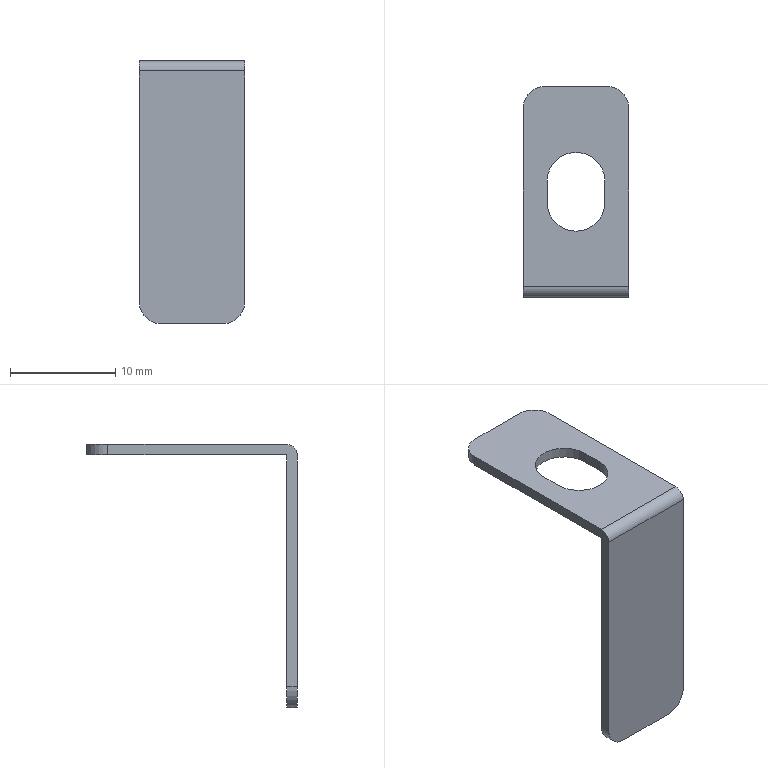Component | SolidWorks | BearingHousingAssembly-1_SensorPlate3-1 | 1 solid | 18 faces | box 10 x 20 x 25 mm | volume 400 mm3 | plane 10 | cylinder 8 | commonest cylinder face diameters 4 x4 5.5 x3 2 x1 | material Plain Carbon Steel
build123d program:
from build123d import *

# Parameters (mm, degrees)
EXTRUDE_THIN1_DEPTH = 5
FILLET1_R           = 1
FILLET2_R           = 2
CUT_EXTRUDE1_DEPTH  = 33.404


with BuildPart() as part:
    # Sketch1 → Extrude-Thin1 (new, symmetric)
    with BuildSketch(Plane.XY):
        Polygon((0, 20), (0, 0), (25, 0), (25, 1), (1, 1), (1, 20), align=None)
    extrude(amount=EXTRUDE_THIN1_DEPTH, both=True)

    # Fillet1
    fillet1_edges = [part.edges().sort_by_distance(p)[0] for p in [
        (0, 0, 0),
    ]]
    fillet(fillet1_edges, radius=FILLET1_R)

    # Fillet2
    fillet2_edges = [part.edges().sort_by_distance(p)[0] for p in [
        (0.5, 20, 5),
        (0.5, 20, -5),
        (25, 0.5, -5),
        (25, 0.5, 5),
    ]]
    fillet(fillet2_edges, radius=FILLET2_R)

    # Sketch2 → Cut-Extrude1 (cut, through all)
    with BuildSketch(Plane.ZY):
        with BuildLine():
            Line((-2.75, 9), (-2.75, 11))
            ThreePointArc((-2.75, 11), (0, 13.75), (2.75, 11))
            Line((2.75, 11), (2.75, 9))
            ThreePointArc((2.75, 9), (0, 6.25), (-2.75, 9))
        make_face()
    extrude(amount=-CUT_EXTRUDE1_DEPTH, mode=Mode.SUBTRACT)


solid = part.part

# Placed as in the assembly
solid = solid.moved(Location((-81.666, 41.264, -46), (0, 90, 0)))
STEP:
#1=COLOUR_RGB('',0.7922,0.8196,0.9333);
#2=FILL_AREA_STYLE_COLOUR('',#1);
#3=FILL_AREA_STYLE('',(#2));
#4=SURFACE_STYLE_FILL_AREA(#3);
#5=SURFACE_SIDE_STYLE('',(#4));
#6=SURFACE_STYLE_USAGE(.BOTH.,#5);
#7=PRESENTATION_STYLE_ASSIGNMENT((#6));
#8=CARTESIAN_POINT('',(-3.107,1.979,-1.85));
#9=VERTEX_POINT('',#8);
#10=CARTESIAN_POINT('',(-3.215,1.871,-1.85));
#11=VERTEX_POINT('',#10);
#12=CARTESIAN_POINT('',(-3.215,1.979,-1.85));
#13=DIRECTION('',(-0.,-0.,-1.));
#14=DIRECTION('',(0.,1.,0.));
#15=AXIS2_PLACEMENT_3D('',#12,#13,#14);
#16=CIRCLE('',#15,0.1083);
#17=EDGE_CURVE('',#9,#11,#16,.T.);
#18=ORIENTED_EDGE('',*,*,#17,.T.);
#19=CARTESIAN_POINT('',(-3.215,1.871,-1.811));
#20=VERTEX_POINT('',#19);
#21=CARTESIAN_POINT('',(-3.215,1.871,-2.795));
#22=DIRECTION('',(0.,0.,1.));
#23=VECTOR('',#22,39.37);
#24=LINE('',#21,#23);
#25=EDGE_CURVE('',#11,#20,#24,.T.);
#26=ORIENTED_EDGE('',*,*,#25,.T.);
#27=CARTESIAN_POINT('',(-3.107,1.979,-1.811));
#28=VERTEX_POINT('',#27);
#29=CARTESIAN_POINT('',(-3.215,1.979,-1.811));
#30=DIRECTION('',(0.,0.,1.));
#31=DIRECTION('',(0.,-1.,0.));
#32=AXIS2_PLACEMENT_3D('',#29,#30,#31);
#33=CIRCLE('',#32,0.1083);
#34=EDGE_CURVE('',#20,#28,#33,.T.);
#35=ORIENTED_EDGE('',*,*,#34,.T.);
#36=CARTESIAN_POINT('',(-3.107,1.979,-2.795));
#37=DIRECTION('',(0.,0.,1.));
#38=VECTOR('',#37,39.37);
#39=LINE('',#36,#38);
#40=EDGE_CURVE('',#9,#28,#39,.T.);
#41=ORIENTED_EDGE('',*,*,#40,.F.);
#42=EDGE_LOOP('',(#18,#26,#35,#41));
#43=FACE_OUTER_BOUND('',#42,.T.);
#44=CARTESIAN_POINT('',(-3.215,1.979,-2.795));
#45=DIRECTION('',(0.,0.,1.));
#46=DIRECTION('',(0.,-1.,0.));
#47=AXIS2_PLACEMENT_3D('',#44,#45,#46);
#48=CYLINDRICAL_SURFACE('',#47,0.1083);
#49=ADVANCED_FACE('',(#43),#48,.F.);
#50=CARTESIAN_POINT('',(-3.412,1.625,-1.85));
#51=VERTEX_POINT('',#50);
#52=CARTESIAN_POINT('',(-3.412,1.625,-2.717));
#53=VERTEX_POINT('',#52);
#54=CARTESIAN_POINT('',(-3.412,1.625,-1.811));
#55=DIRECTION('',(-0.,0.,-1.));
#56=VECTOR('',#55,39.37);
#57=LINE('',#54,#56);
#58=EDGE_CURVE('',#51,#53,#57,.T.);
#59=ORIENTED_EDGE('',*,*,#58,.T.);
#60=CARTESIAN_POINT('',(-3.333,1.625,-2.795));
#61=VERTEX_POINT('',#60);
#62=CARTESIAN_POINT('',(-3.333,1.625,-2.717));
#63=DIRECTION('',(-0.,-1.,-0.));
#64=DIRECTION('',(1.,0.,-0.));
#65=AXIS2_PLACEMENT_3D('',#62,#63,#64);
#66=CIRCLE('',#65,0.07874);
#67=EDGE_CURVE('',#53,#61,#66,.T.);
#68=ORIENTED_EDGE('',*,*,#67,.T.);
#69=CARTESIAN_POINT('',(-3.097,1.625,-2.795));
#70=VERTEX_POINT('',#69);
#71=CARTESIAN_POINT('',(-3.018,1.625,-2.795));
#72=DIRECTION('',(-1.,0.,0.));
#73=VECTOR('',#72,39.37);
#74=LINE('',#71,#73);
#75=EDGE_CURVE('',#70,#61,#74,.T.);
#76=ORIENTED_EDGE('',*,*,#75,.F.);
#77=CARTESIAN_POINT('',(-3.018,1.625,-2.717));
#78=VERTEX_POINT('',#77);
#79=CARTESIAN_POINT('',(-3.097,1.625,-2.717));
#80=DIRECTION('',(-0.,-1.,-0.));
#81=DIRECTION('',(1.,0.,-0.));
#82=AXIS2_PLACEMENT_3D('',#79,#80,#81);
#83=CIRCLE('',#82,0.07874);
#84=EDGE_CURVE('',#70,#78,#83,.T.);
#85=ORIENTED_EDGE('',*,*,#84,.T.);
#86=CARTESIAN_POINT('',(-3.018,1.625,-1.85));
#87=VERTEX_POINT('',#86);
#88=CARTESIAN_POINT('',(-3.018,1.625,-1.811));
#89=DIRECTION('',(-0.,0.,-1.));
#90=VECTOR('',#89,39.37);
#91=LINE('',#88,#90);
#92=EDGE_CURVE('',#87,#78,#91,.T.);
#93=ORIENTED_EDGE('',*,*,#92,.F.);
#94=CARTESIAN_POINT('',(-3.018,1.625,-1.85));
#95=DIRECTION('',(-1.,0.,0.));
#96=VECTOR('',#95,39.37);
#97=LINE('',#94,#96);
#98=EDGE_CURVE('',#87,#51,#97,.T.);
#99=ORIENTED_EDGE('',*,*,#98,.T.);
#100=EDGE_LOOP('',(#59,#68,#76,#85,#93,#99));
#101=FACE_OUTER_BOUND('',#100,.T.);
#102=CARTESIAN_POINT('',(-3.018,1.625,-1.811));
#103=DIRECTION('',(0.,1.,0.));
#104=DIRECTION('',(1.,-0.,-0.));
#105=AXIS2_PLACEMENT_3D('',#102,#103,#104);
#106=PLANE('',#105);
#107=ADVANCED_FACE('',(#101),#106,.F.);
#108=ORIENTED_EDGE('',*,*,#75,.T.);
#109=CARTESIAN_POINT('',(-3.333,1.664,-2.795));
#110=VERTEX_POINT('',#109);
#111=CARTESIAN_POINT('',(-3.333,1.664,-2.795));
#112=DIRECTION('',(0.,1.,0.));
#113=VECTOR('',#112,39.37);
#114=LINE('',#111,#113);
#115=EDGE_CURVE('',#61,#110,#114,.T.);
#116=ORIENTED_EDGE('',*,*,#115,.T.);
#117=CARTESIAN_POINT('',(-3.097,1.664,-2.795));
#118=VERTEX_POINT('',#117);
#119=CARTESIAN_POINT('',(-3.018,1.664,-2.795));
#120=DIRECTION('',(-1.,0.,0.));
#121=VECTOR('',#120,39.37);
#122=LINE('',#119,#121);
#123=EDGE_CURVE('',#118,#110,#122,.T.);
#124=ORIENTED_EDGE('',*,*,#123,.F.);
#125=CARTESIAN_POINT('',(-3.097,1.625,-2.795));
#126=DIRECTION('',(-0.,-1.,-0.));
#127=VECTOR('',#126,39.37);
#128=LINE('',#125,#127);
#129=EDGE_CURVE('',#118,#70,#128,.T.);
#130=ORIENTED_EDGE('',*,*,#129,.T.);
#131=EDGE_LOOP('',(#108,#116,#124,#130));
#132=FACE_OUTER_BOUND('',#131,.T.);
#133=CARTESIAN_POINT('',(-3.018,1.664,-2.795));
#134=DIRECTION('',(-0.,0.,-1.));
#135=DIRECTION('',(-1.,0.,0.));
#136=AXIS2_PLACEMENT_3D('',#133,#134,#135);
#137=PLANE('',#136);
#138=ADVANCED_FACE('',(#132),#137,.T.);
#139=ORIENTED_EDGE('',*,*,#123,.T.);
#140=CARTESIAN_POINT('',(-3.412,1.664,-2.717));
#141=VERTEX_POINT('',#140);
#142=CARTESIAN_POINT('',(-3.333,1.664,-2.717));
#143=DIRECTION('',(0.,1.,0.));
#144=DIRECTION('',(1.,0.,-0.));
#145=AXIS2_PLACEMENT_3D('',#142,#143,#144);
#146=CIRCLE('',#145,0.07874);
#147=EDGE_CURVE('',#110,#141,#146,.T.);
#148=ORIENTED_EDGE('',*,*,#147,.T.);
#149=CARTESIAN_POINT('',(-3.412,1.664,-1.85));
#150=VERTEX_POINT('',#149);
#151=CARTESIAN_POINT('',(-3.412,1.664,-1.811));
#152=DIRECTION('',(-0.,0.,-1.));
#153=VECTOR('',#152,39.37);
#154=LINE('',#151,#153);
#155=EDGE_CURVE('',#150,#141,#154,.T.);
#156=ORIENTED_EDGE('',*,*,#155,.F.);
#157=CARTESIAN_POINT('',(-3.018,1.664,-1.85));
#158=VERTEX_POINT('',#157);
#159=CARTESIAN_POINT('',(-3.018,1.664,-1.85));
#160=DIRECTION('',(-1.,0.,0.));
#161=VECTOR('',#160,39.37);
#162=LINE('',#159,#161);
#163=EDGE_CURVE('',#158,#150,#162,.T.);
#164=ORIENTED_EDGE('',*,*,#163,.F.);
#165=CARTESIAN_POINT('',(-3.018,1.664,-2.717));
#166=VERTEX_POINT('',#165);
#167=CARTESIAN_POINT('',(-3.018,1.664,-1.811));
#168=DIRECTION('',(-0.,0.,-1.));
#169=VECTOR('',#168,39.37);
#170=LINE('',#167,#169);
#171=EDGE_CURVE('',#158,#166,#170,.T.);
#172=ORIENTED_EDGE('',*,*,#171,.T.);
#173=CARTESIAN_POINT('',(-3.097,1.664,-2.717));
#174=DIRECTION('',(0.,1.,0.));
#175=DIRECTION('',(1.,0.,-0.));
#176=AXIS2_PLACEMENT_3D('',#173,#174,#175);
#177=CIRCLE('',#176,0.07874);
#178=EDGE_CURVE('',#166,#118,#177,.T.);
#179=ORIENTED_EDGE('',*,*,#178,.T.);
#180=EDGE_LOOP('',(#139,#148,#156,#164,#172,#179));
#181=FACE_OUTER_BOUND('',#180,.T.);
#182=CARTESIAN_POINT('',(-3.018,1.664,-1.811));
#183=DIRECTION('',(0.,1.,0.));
#184=DIRECTION('',(1.,-0.,-0.));
#185=AXIS2_PLACEMENT_3D('',#182,#183,#184);
#186=PLANE('',#185);
#187=ADVANCED_FACE('',(#181),#186,.T.);
#188=ORIENTED_EDGE('',*,*,#17,.F.);
#189=CARTESIAN_POINT('',(-3.107,2.058,-1.85));
#190=VERTEX_POINT('',#189);
#191=CARTESIAN_POINT('',(-3.107,2.412,-1.85));
#192=DIRECTION('',(0.,-1.,0.));
#193=VECTOR('',#192,39.37);
#194=LINE('',#191,#193);
#195=EDGE_CURVE('',#190,#9,#194,.T.);
#196=ORIENTED_EDGE('',*,*,#195,.F.);
#197=CARTESIAN_POINT('',(-3.323,2.058,-1.85));
#198=VERTEX_POINT('',#197);
#199=CARTESIAN_POINT('',(-3.215,2.058,-1.85));
#200=DIRECTION('',(-0.,-0.,-1.));
#201=DIRECTION('',(0.,1.,0.));
#202=AXIS2_PLACEMENT_3D('',#199,#200,#201);
#203=CIRCLE('',#202,0.1083);
#204=EDGE_CURVE('',#198,#190,#203,.T.);
#205=ORIENTED_EDGE('',*,*,#204,.F.);
#206=CARTESIAN_POINT('',(-3.323,1.979,-1.85));
#207=VERTEX_POINT('',#206);
#208=CARTESIAN_POINT('',(-3.323,2.412,-1.85));
#209=DIRECTION('',(-0.,1.,-0.));
#210=VECTOR('',#209,39.37);
#211=LINE('',#208,#210);
#212=EDGE_CURVE('',#207,#198,#211,.T.);
#213=ORIENTED_EDGE('',*,*,#212,.F.);
#214=CARTESIAN_POINT('',(-3.215,1.979,-1.85));
#215=DIRECTION('',(-0.,-0.,-1.));
#216=DIRECTION('',(0.,1.,0.));
#217=AXIS2_PLACEMENT_3D('',#214,#215,#216);
#218=CIRCLE('',#217,0.1083);
#219=EDGE_CURVE('',#11,#207,#218,.T.);
#220=ORIENTED_EDGE('',*,*,#219,.F.);
#221=EDGE_LOOP('',(#188,#196,#205,#213,#220));
#222=FACE_BOUND('',#221,.T.);
#223=CARTESIAN_POINT('',(-3.412,2.333,-1.85));
#224=VERTEX_POINT('',#223);
#225=CARTESIAN_POINT('',(-3.412,2.412,-1.85));
#226=DIRECTION('',(-0.,-1.,0.));
#227=VECTOR('',#226,39.37);
#228=LINE('',#225,#227);
#229=EDGE_CURVE('',#224,#150,#228,.T.);
#230=ORIENTED_EDGE('',*,*,#229,.F.);
#231=CARTESIAN_POINT('',(-3.333,2.412,-1.85));
#232=VERTEX_POINT('',#231);
#233=CARTESIAN_POINT('',(-3.333,2.333,-1.85));
#234=DIRECTION('',(-0.,-0.,-1.));
#235=DIRECTION('',(0.,1.,0.));
#236=AXIS2_PLACEMENT_3D('',#233,#234,#235);
#237=CIRCLE('',#236,0.07874);
#238=EDGE_CURVE('',#224,#232,#237,.T.);
#239=ORIENTED_EDGE('',*,*,#238,.T.);
#240=CARTESIAN_POINT('',(-3.097,2.412,-1.85));
#241=VERTEX_POINT('',#240);
#242=CARTESIAN_POINT('',(-3.018,2.412,-1.85));
#243=DIRECTION('',(-1.,0.,0.));
#244=VECTOR('',#243,39.37);
#245=LINE('',#242,#244);
#246=EDGE_CURVE('',#241,#232,#245,.T.);
#247=ORIENTED_EDGE('',*,*,#246,.F.);
#248=CARTESIAN_POINT('',(-3.018,2.333,-1.85));
#249=VERTEX_POINT('',#248);
#250=CARTESIAN_POINT('',(-3.097,2.333,-1.85));
#251=DIRECTION('',(-0.,-0.,-1.));
#252=DIRECTION('',(0.,1.,0.));
#253=AXIS2_PLACEMENT_3D('',#250,#251,#252);
#254=CIRCLE('',#253,0.07874);
#255=EDGE_CURVE('',#241,#249,#254,.T.);
#256=ORIENTED_EDGE('',*,*,#255,.T.);
#257=CARTESIAN_POINT('',(-3.018,2.412,-1.85));
#258=DIRECTION('',(-0.,-1.,0.));
#259=VECTOR('',#258,39.37);
#260=LINE('',#257,#259);
#261=EDGE_CURVE('',#249,#158,#260,.T.);
#262=ORIENTED_EDGE('',*,*,#261,.T.);
#263=ORIENTED_EDGE('',*,*,#163,.T.);
#264=EDGE_LOOP('',(#230,#239,#247,#256,#262,#263));
#265=FACE_OUTER_BOUND('',#264,.T.);
#266=CARTESIAN_POINT('',(-3.018,2.412,-1.85));
#267=DIRECTION('',(-0.,-0.,-1.));
#268=DIRECTION('',(0.,1.,-0.));
#269=AXIS2_PLACEMENT_3D('',#266,#267,#268);
#270=PLANE('',#269);
#271=ADVANCED_FACE('',(#222,#265),#270,.T.);
#272=ORIENTED_EDGE('',*,*,#246,.T.);
#273=CARTESIAN_POINT('',(-3.333,2.412,-1.811));
#274=VERTEX_POINT('',#273);
#275=CARTESIAN_POINT('',(-3.333,2.412,-1.811));
#276=DIRECTION('',(0.,-0.,1.));
#277=VECTOR('',#276,39.37);
#278=LINE('',#275,#277);
#279=EDGE_CURVE('',#232,#274,#278,.T.);
#280=ORIENTED_EDGE('',*,*,#279,.T.);
#281=CARTESIAN_POINT('',(-3.097,2.412,-1.811));
#282=VERTEX_POINT('',#281);
#283=CARTESIAN_POINT('',(-3.018,2.412,-1.811));
#284=DIRECTION('',(-1.,0.,0.));
#285=VECTOR('',#284,39.37);
#286=LINE('',#283,#285);
#287=EDGE_CURVE('',#282,#274,#286,.T.);
#288=ORIENTED_EDGE('',*,*,#287,.F.);
#289=CARTESIAN_POINT('',(-3.097,2.412,-1.85));
#290=DIRECTION('',(-0.,0.,-1.));
#291=VECTOR('',#290,39.37);
#292=LINE('',#289,#291);
#293=EDGE_CURVE('',#282,#241,#292,.T.);
#294=ORIENTED_EDGE('',*,*,#293,.T.);
#295=EDGE_LOOP('',(#272,#280,#288,#294));
#296=FACE_OUTER_BOUND('',#295,.T.);
#297=CARTESIAN_POINT('',(-3.018,2.412,-1.811));
#298=DIRECTION('',(0.,1.,0.));
#299=DIRECTION('',(1.,-0.,-0.));
#300=AXIS2_PLACEMENT_3D('',#297,#298,#299);
#301=PLANE('',#300);
#302=ADVANCED_FACE('',(#296),#301,.T.);
#303=CARTESIAN_POINT('',(-3.107,2.058,-1.811));
#304=VERTEX_POINT('',#303);
#305=CARTESIAN_POINT('',(-3.107,1.979,-1.811));
#306=DIRECTION('',(-0.,1.,-0.));
#307=VECTOR('',#306,39.37);
#308=LINE('',#305,#307);
#309=EDGE_CURVE('',#28,#304,#308,.T.);
#310=ORIENTED_EDGE('',*,*,#309,.F.);
#311=ORIENTED_EDGE('',*,*,#34,.F.);
#312=CARTESIAN_POINT('',(-3.323,1.979,-1.811));
#313=VERTEX_POINT('',#312);
#314=CARTESIAN_POINT('',(-3.215,1.979,-1.811));
#315=DIRECTION('',(0.,0.,1.));
#316=DIRECTION('',(0.,-1.,0.));
#317=AXIS2_PLACEMENT_3D('',#314,#315,#316);
#318=CIRCLE('',#317,0.1083);
#319=EDGE_CURVE('',#313,#20,#318,.T.);
#320=ORIENTED_EDGE('',*,*,#319,.F.);
#321=CARTESIAN_POINT('',(-3.323,2.058,-1.811));
#322=VERTEX_POINT('',#321);
#323=CARTESIAN_POINT('',(-3.323,1.979,-1.811));
#324=DIRECTION('',(0.,-1.,0.));
#325=VECTOR('',#324,39.37);
#326=LINE('',#323,#325);
#327=EDGE_CURVE('',#322,#313,#326,.T.);
#328=ORIENTED_EDGE('',*,*,#327,.F.);
#329=CARTESIAN_POINT('',(-3.215,2.058,-1.811));
#330=DIRECTION('',(0.,0.,1.));
#331=DIRECTION('',(0.,-1.,0.));
#332=AXIS2_PLACEMENT_3D('',#329,#330,#331);
#333=CIRCLE('',#332,0.1083);
#334=EDGE_CURVE('',#304,#322,#333,.T.);
#335=ORIENTED_EDGE('',*,*,#334,.F.);
#336=EDGE_LOOP('',(#310,#311,#320,#328,#335));
#337=FACE_BOUND('',#336,.T.);
#338=ORIENTED_EDGE('',*,*,#287,.T.);
#339=CARTESIAN_POINT('',(-3.412,2.333,-1.811));
#340=VERTEX_POINT('',#339);
#341=CARTESIAN_POINT('',(-3.333,2.333,-1.811));
#342=DIRECTION('',(0.,0.,1.));
#343=DIRECTION('',(0.,1.,0.));
#344=AXIS2_PLACEMENT_3D('',#341,#342,#343);
#345=CIRCLE('',#344,0.07874);
#346=EDGE_CURVE('',#274,#340,#345,.T.);
#347=ORIENTED_EDGE('',*,*,#346,.T.);
#348=CARTESIAN_POINT('',(-3.412,1.664,-1.811));
#349=VERTEX_POINT('',#348);
#350=CARTESIAN_POINT('',(-3.412,2.412,-1.811));
#351=DIRECTION('',(-0.,-1.,0.));
#352=VECTOR('',#351,39.37);
#353=LINE('',#350,#352);
#354=EDGE_CURVE('',#340,#349,#353,.T.);
#355=ORIENTED_EDGE('',*,*,#354,.T.);
#356=CARTESIAN_POINT('',(-3.018,1.664,-1.811));
#357=VERTEX_POINT('',#356);
#358=CARTESIAN_POINT('',(-3.018,1.664,-1.811));
#359=DIRECTION('',(1.,-0.,-0.));
#360=VECTOR('',#359,39.37);
#361=LINE('',#358,#360);
#362=EDGE_CURVE('',#349,#357,#361,.T.);
#363=ORIENTED_EDGE('',*,*,#362,.T.);
#364=CARTESIAN_POINT('',(-3.018,2.333,-1.811));
#365=VERTEX_POINT('',#364);
#366=CARTESIAN_POINT('',(-3.018,2.412,-1.811));
#367=DIRECTION('',(-0.,-1.,0.));
#368=VECTOR('',#367,39.37);
#369=LINE('',#366,#368);
#370=EDGE_CURVE('',#365,#357,#369,.T.);
#371=ORIENTED_EDGE('',*,*,#370,.F.);
#372=CARTESIAN_POINT('',(-3.097,2.333,-1.811));
#373=DIRECTION('',(0.,0.,1.));
#374=DIRECTION('',(0.,1.,0.));
#375=AXIS2_PLACEMENT_3D('',#372,#373,#374);
#376=CIRCLE('',#375,0.07874);
#377=EDGE_CURVE('',#365,#282,#376,.T.);
#378=ORIENTED_EDGE('',*,*,#377,.T.);
#379=EDGE_LOOP('',(#338,#347,#355,#363,#371,#378));
#380=FACE_OUTER_BOUND('',#379,.T.);
#381=CARTESIAN_POINT('',(-3.018,2.412,-1.811));
#382=DIRECTION('',(-0.,-0.,-1.));
#383=DIRECTION('',(0.,1.,-0.));
#384=AXIS2_PLACEMENT_3D('',#381,#382,#383);
#385=PLANE('',#384);
#386=ADVANCED_FACE('',(#337,#380),#385,.F.);
#387=ORIENTED_EDGE('',*,*,#261,.F.);
#388=CARTESIAN_POINT('',(-3.018,2.333,-1.811));
#389=DIRECTION('',(0.,-0.,1.));
#390=VECTOR('',#389,39.37);
#391=LINE('',#388,#390);
#392=EDGE_CURVE('',#249,#365,#391,.T.);
#393=ORIENTED_EDGE('',*,*,#392,.T.);
#394=ORIENTED_EDGE('',*,*,#370,.T.);
#395=CARTESIAN_POINT('',(-3.018,1.664,-1.85));
#396=DIRECTION('',(1.,-0.,-0.));
#397=DIRECTION('',(0.,0.,1.));
#398=AXIS2_PLACEMENT_3D('',#395,#396,#397);
#399=CIRCLE('',#398,0.03937);
#400=EDGE_CURVE('',#357,#87,#399,.T.);
#401=ORIENTED_EDGE('',*,*,#400,.T.);
#402=ORIENTED_EDGE('',*,*,#92,.T.);
#403=CARTESIAN_POINT('',(-3.018,1.664,-2.717));
#404=DIRECTION('',(0.,1.,0.));
#405=VECTOR('',#404,39.37);
#406=LINE('',#403,#405);
#407=EDGE_CURVE('',#78,#166,#406,.T.);
#408=ORIENTED_EDGE('',*,*,#407,.T.);
#409=ORIENTED_EDGE('',*,*,#171,.F.);
#410=EDGE_LOOP('',(#387,#393,#394,#401,#402,#408,#409));
#411=FACE_OUTER_BOUND('',#410,.T.);
#412=CARTESIAN_POINT('',(-3.018,1.625,-1.811));
#413=DIRECTION('',(-1.,0.,0.));
#414=DIRECTION('',(0.,-0.,1.));
#415=AXIS2_PLACEMENT_3D('',#412,#413,#414);
#416=PLANE('',#415);
#417=ADVANCED_FACE('',(#411),#416,.F.);
#418=ORIENTED_EDGE('',*,*,#354,.F.);
#419=CARTESIAN_POINT('',(-3.412,2.333,-1.811));
#420=DIRECTION('',(-0.,0.,-1.));
#421=VECTOR('',#420,39.37);
#422=LINE('',#419,#421);
#423=EDGE_CURVE('',#340,#224,#422,.T.);
#424=ORIENTED_EDGE('',*,*,#423,.T.);
#425=ORIENTED_EDGE('',*,*,#229,.T.);
#426=ORIENTED_EDGE('',*,*,#155,.T.);
#427=CARTESIAN_POINT('',(-3.412,1.625,-2.717));
#428=DIRECTION('',(-0.,-1.,-0.));
#429=VECTOR('',#428,39.37);
#430=LINE('',#427,#429);
#431=EDGE_CURVE('',#141,#53,#430,.T.);
#432=ORIENTED_EDGE('',*,*,#431,.T.);
#433=ORIENTED_EDGE('',*,*,#58,.F.);
#434=CARTESIAN_POINT('',(-3.412,1.664,-1.85));
#435=DIRECTION('',(-1.,0.,0.));
#436=DIRECTION('',(0.,0.,1.));
#437=AXIS2_PLACEMENT_3D('',#434,#435,#436);
#438=CIRCLE('',#437,0.03937);
#439=EDGE_CURVE('',#51,#349,#438,.T.);
#440=ORIENTED_EDGE('',*,*,#439,.T.);
#441=EDGE_LOOP('',(#418,#424,#425,#426,#432,#433,#440));
#442=FACE_OUTER_BOUND('',#441,.T.);
#443=CARTESIAN_POINT('',(-3.412,1.625,-1.811));
#444=DIRECTION('',(-1.,0.,0.));
#445=DIRECTION('',(0.,-0.,1.));
#446=AXIS2_PLACEMENT_3D('',#443,#444,#445);
#447=PLANE('',#446);
#448=ADVANCED_FACE('',(#442),#447,.T.);
#449=ORIENTED_EDGE('',*,*,#400,.F.);
#450=ORIENTED_EDGE('',*,*,#362,.F.);
#451=ORIENTED_EDGE('',*,*,#439,.F.);
#452=ORIENTED_EDGE('',*,*,#98,.F.);
#453=EDGE_LOOP('',(#449,#450,#451,#452));
#454=FACE_OUTER_BOUND('',#453,.T.);
#455=CARTESIAN_POINT('',(-3.018,1.664,-1.85));
#456=DIRECTION('',(-1.,0.,0.));
#457=DIRECTION('',(0.,0.,1.));
#458=AXIS2_PLACEMENT_3D('',#455,#456,#457);
#459=CYLINDRICAL_SURFACE('',#458,0.03937);
#460=ADVANCED_FACE('',(#454),#459,.T.);
#461=ORIENTED_EDGE('',*,*,#346,.F.);
#462=ORIENTED_EDGE('',*,*,#279,.F.);
#463=ORIENTED_EDGE('',*,*,#238,.F.);
#464=ORIENTED_EDGE('',*,*,#423,.F.);
#465=EDGE_LOOP('',(#461,#462,#463,#464));
#466=FACE_OUTER_BOUND('',#465,.T.);
#467=CARTESIAN_POINT('',(-3.333,2.333,-1.811));
#468=DIRECTION('',(-0.,0.,-1.));
#469=DIRECTION('',(-1.,0.,0.));
#470=AXIS2_PLACEMENT_3D('',#467,#468,#469);
#471=CYLINDRICAL_SURFACE('',#470,0.07874);
#472=ADVANCED_FACE('',(#466),#471,.T.);
#473=ORIENTED_EDGE('',*,*,#377,.F.);
#474=ORIENTED_EDGE('',*,*,#392,.F.);
#475=ORIENTED_EDGE('',*,*,#255,.F.);
#476=ORIENTED_EDGE('',*,*,#293,.F.);
#477=EDGE_LOOP('',(#473,#474,#475,#476));
#478=FACE_OUTER_BOUND('',#477,.T.);
#479=CARTESIAN_POINT('',(-3.097,2.333,-1.811));
#480=DIRECTION('',(0.,-0.,1.));
#481=DIRECTION('',(1.,0.,-0.));
#482=AXIS2_PLACEMENT_3D('',#479,#480,#481);
#483=CYLINDRICAL_SURFACE('',#482,0.07874);
#484=ADVANCED_FACE('',(#478),#483,.T.);
#485=ORIENTED_EDGE('',*,*,#147,.F.);
#486=ORIENTED_EDGE('',*,*,#115,.F.);
#487=ORIENTED_EDGE('',*,*,#67,.F.);
#488=ORIENTED_EDGE('',*,*,#431,.F.);
#489=EDGE_LOOP('',(#485,#486,#487,#488));
#490=FACE_OUTER_BOUND('',#489,.T.);
#491=CARTESIAN_POINT('',(-3.333,1.625,-2.717));
#492=DIRECTION('',(-0.,-1.,-0.));
#493=DIRECTION('',(-1.,0.,0.));
#494=AXIS2_PLACEMENT_3D('',#491,#492,#493);
#495=CYLINDRICAL_SURFACE('',#494,0.07874);
#496=ADVANCED_FACE('',(#490),#495,.T.);
#497=ORIENTED_EDGE('',*,*,#178,.F.);
#498=ORIENTED_EDGE('',*,*,#407,.F.);
#499=ORIENTED_EDGE('',*,*,#84,.F.);
#500=ORIENTED_EDGE('',*,*,#129,.F.);
#501=EDGE_LOOP('',(#497,#498,#499,#500));
#502=FACE_OUTER_BOUND('',#501,.T.);
#503=CARTESIAN_POINT('',(-3.097,1.664,-2.717));
#504=DIRECTION('',(0.,1.,0.));
#505=DIRECTION('',(1.,0.,-0.));
#506=AXIS2_PLACEMENT_3D('',#503,#504,#505);
#507=CYLINDRICAL_SURFACE('',#506,0.07874);
#508=ADVANCED_FACE('',(#502),#507,.T.);
#509=ORIENTED_EDGE('',*,*,#25,.F.);
#510=ORIENTED_EDGE('',*,*,#219,.T.);
#511=CARTESIAN_POINT('',(-3.323,1.979,-2.795));
#512=DIRECTION('',(0.,0.,1.));
#513=VECTOR('',#512,39.37);
#514=LINE('',#511,#513);
#515=EDGE_CURVE('',#207,#313,#514,.T.);
#516=ORIENTED_EDGE('',*,*,#515,.T.);
#517=ORIENTED_EDGE('',*,*,#319,.T.);
#518=EDGE_LOOP('',(#509,#510,#516,#517));
#519=FACE_OUTER_BOUND('',#518,.T.);
#520=CARTESIAN_POINT('',(-3.215,1.979,-2.795));
#521=DIRECTION('',(0.,0.,1.));
#522=DIRECTION('',(0.,-1.,0.));
#523=AXIS2_PLACEMENT_3D('',#520,#521,#522);
#524=CYLINDRICAL_SURFACE('',#523,0.1083);
#525=ADVANCED_FACE('',(#519),#524,.F.);
#526=ORIENTED_EDGE('',*,*,#212,.T.);
#527=CARTESIAN_POINT('',(-3.323,2.058,-2.795));
#528=DIRECTION('',(0.,0.,1.));
#529=VECTOR('',#528,39.37);
#530=LINE('',#527,#529);
#531=EDGE_CURVE('',#198,#322,#530,.T.);
#532=ORIENTED_EDGE('',*,*,#531,.T.);
#533=ORIENTED_EDGE('',*,*,#327,.T.);
#534=ORIENTED_EDGE('',*,*,#515,.F.);
#535=EDGE_LOOP('',(#526,#532,#533,#534));
#536=FACE_OUTER_BOUND('',#535,.T.);
#537=CARTESIAN_POINT('',(-3.323,1.979,-2.795));
#538=DIRECTION('',(-1.,-0.,0.));
#539=DIRECTION('',(-0.,1.,0.));
#540=AXIS2_PLACEMENT_3D('',#537,#538,#539);
#541=PLANE('',#540);
#542=ADVANCED_FACE('',(#536),#541,.F.);
#543=ORIENTED_EDGE('',*,*,#204,.T.);
#544=CARTESIAN_POINT('',(-3.107,2.058,-2.795));
#545=DIRECTION('',(0.,0.,1.));
#546=VECTOR('',#545,39.37);
#547=LINE('',#544,#546);
#548=EDGE_CURVE('',#190,#304,#547,.T.);
#549=ORIENTED_EDGE('',*,*,#548,.T.);
#550=ORIENTED_EDGE('',*,*,#334,.T.);
#551=ORIENTED_EDGE('',*,*,#531,.F.);
#552=EDGE_LOOP('',(#543,#549,#550,#551));
#553=FACE_OUTER_BOUND('',#552,.T.);
#554=CARTESIAN_POINT('',(-3.215,2.058,-2.795));
#555=DIRECTION('',(0.,0.,1.));
#556=DIRECTION('',(0.,-1.,0.));
#557=AXIS2_PLACEMENT_3D('',#554,#555,#556);
#558=CYLINDRICAL_SURFACE('',#557,0.1083);
#559=ADVANCED_FACE('',(#553),#558,.F.);
#560=ORIENTED_EDGE('',*,*,#195,.T.);
#561=ORIENTED_EDGE('',*,*,#40,.T.);
#562=ORIENTED_EDGE('',*,*,#309,.T.);
#563=ORIENTED_EDGE('',*,*,#548,.F.);
#564=EDGE_LOOP('',(#560,#561,#562,#563));
#565=FACE_OUTER_BOUND('',#564,.T.);
#566=CARTESIAN_POINT('',(-3.107,1.979,-2.795));
#567=DIRECTION('',(1.,0.,-0.));
#568=DIRECTION('',(0.,-1.,-0.));
#569=AXIS2_PLACEMENT_3D('',#566,#567,#568);
#570=PLANE('',#569);
#571=ADVANCED_FACE('',(#565),#570,.F.);
#572=CLOSED_SHELL('',(#49,#107,#138,#187,#271,#302,#386,#417,#448,#460,#472,#484,#496,#508,#525,#542,#559,#571));
#573=MANIFOLD_SOLID_BREP('',#572);
#574=STYLED_ITEM('',(#7),#573);
#575=(LENGTH_UNIT()NAMED_UNIT(*)SI_UNIT($,.METRE.));
#576=LENGTH_MEASURE_WITH_UNIT(LENGTH_MEASURE(0.0254),#575);
#577=DIMENSIONAL_EXPONENTS(1.,0.,0.,0.,0.,0.,0.);
#578=(CONVERSION_BASED_UNIT('',#576)LENGTH_UNIT()NAMED_UNIT(#577));
#579=UNCERTAINTY_MEASURE_WITH_UNIT(LENGTH_MEASURE(0.00001),#578,'','');
#580=(NAMED_UNIT(*)PLANE_ANGLE_UNIT()SI_UNIT($,.RADIAN.));
#581=(NAMED_UNIT(*)SI_UNIT($,.STERADIAN.)SOLID_ANGLE_UNIT());
#582=(GEOMETRIC_REPRESENTATION_CONTEXT(3)GLOBAL_UNCERTAINTY_ASSIGNED_CONTEXT((#579))GLOBAL_UNIT_ASSIGNED_CONTEXT((#578,#580,#581))REPRESENTATION_CONTEXT('',''));
#583=MECHANICAL_DESIGN_GEOMETRIC_PRESENTATION_REPRESENTATION('',(#574),#582);
#584=CARTESIAN_POINT('',(0.,0.,0.));
#585=DIRECTION('',(0.,0.,1.));
#586=DIRECTION('',(1.,0.,0.));
#587=AXIS2_PLACEMENT_3D('',#584,#585,#586);
#588=(LENGTH_UNIT()NAMED_UNIT(*)SI_UNIT($,.METRE.));
#589=LENGTH_MEASURE_WITH_UNIT(LENGTH_MEASURE(0.0254),#588);
#590=DIMENSIONAL_EXPONENTS(1.,0.,0.,0.,0.,0.,0.);
#591=(CONVERSION_BASED_UNIT('',#589)LENGTH_UNIT()NAMED_UNIT(#590));
#592=UNCERTAINTY_MEASURE_WITH_UNIT(LENGTH_MEASURE(0.00001),#591,'','');
#593=(NAMED_UNIT(*)PLANE_ANGLE_UNIT()SI_UNIT($,.RADIAN.));
#594=(NAMED_UNIT(*)SI_UNIT($,.STERADIAN.)SOLID_ANGLE_UNIT());
#595=(GEOMETRIC_REPRESENTATION_CONTEXT(3)GLOBAL_UNCERTAINTY_ASSIGNED_CONTEXT((#592))GLOBAL_UNIT_ASSIGNED_CONTEXT((#591,#593,#594))REPRESENTATION_CONTEXT('',''));
#596=ADVANCED_BREP_SHAPE_REPRESENTATION('',(#573,#587),#595);
#597=PRESENTATION_LAYER_ASSIGNMENT('','',(#574));